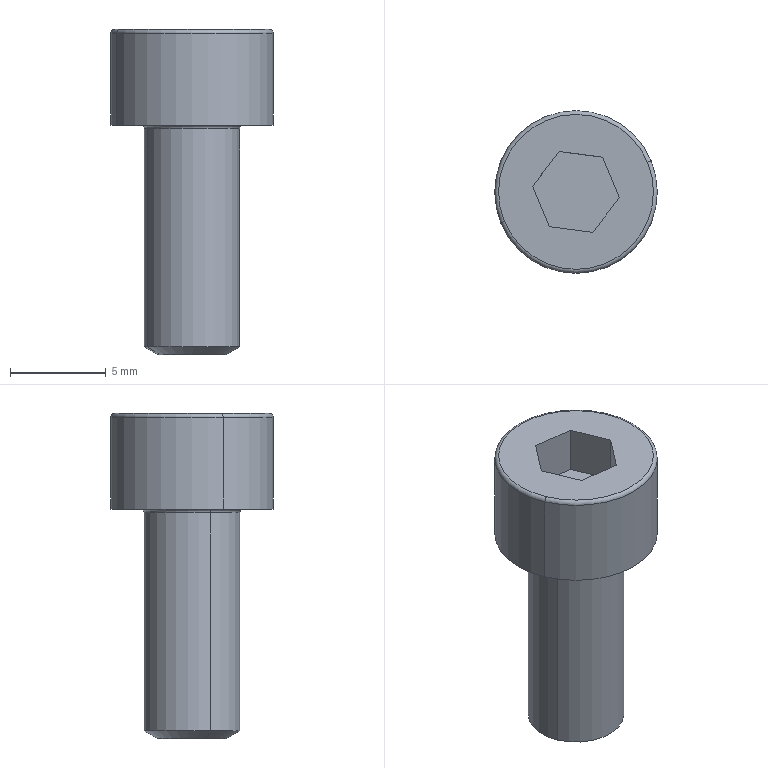Component | NX | HEX_SCREW_M5X12 | 1 solid | 20 faces | volume 483 mm3 | plane 10 | torus 4 | cylinder 4 | cone 2 | commonest cylinder face diameters 8.5 x2 5 x2